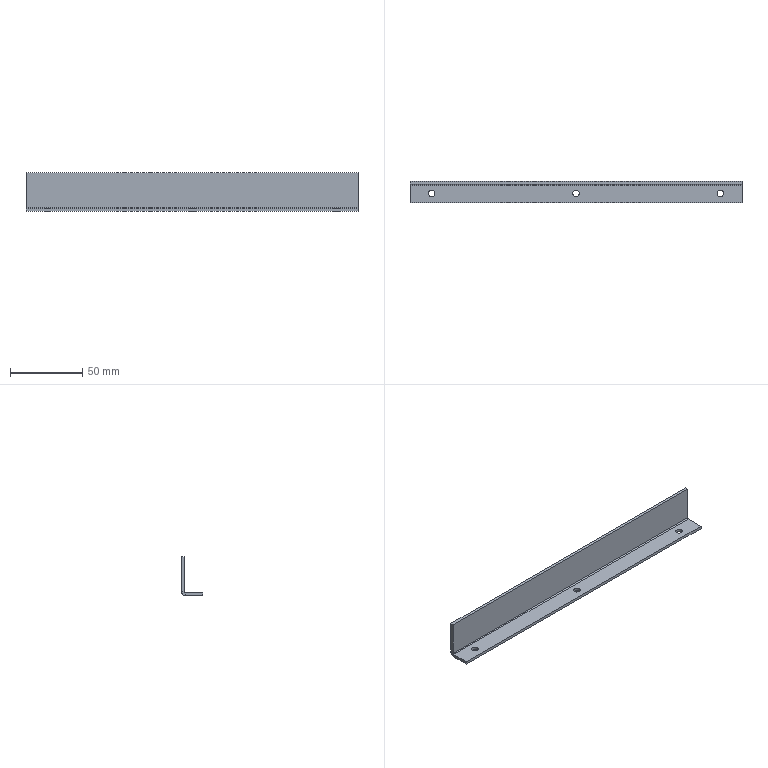Component | SolidWorks | P-SLJ-001-003-2 | 1 solid | 20 faces | box 230 x 15 x 27 mm | volume 17962 mm3 | plane 12 | cylinder 8 | commonest cylinder face diameters 4.5 x6 5.473 x1 1.473 x1 | material SUS 304
STEP:
#1=COLOUR_RGB('',0.7922,0.8196,0.9333);
#2=FILL_AREA_STYLE_COLOUR('',#1);
#3=FILL_AREA_STYLE('',(#2));
#4=SURFACE_STYLE_FILL_AREA(#3);
#5=SURFACE_SIDE_STYLE('',(#4));
#6=SURFACE_STYLE_USAGE(.BOTH.,#5);
#7=PRESENTATION_STYLE_ASSIGNMENT((#6));
#8=CARTESIAN_POINT('',(-1.801,-2.579,39.434));
#9=VERTEX_POINT('',#8);
#10=CARTESIAN_POINT('',(-1.624,-2.579,39.434));
#11=VERTEX_POINT('',#10);
#12=CARTESIAN_POINT('',(-1.713,-2.579,39.434));
#13=DIRECTION('',(0.,0.,1.));
#14=DIRECTION('',(1.,0.,0.));
#15=AXIS2_PLACEMENT_3D('',#12,#13,#14);
#16=CIRCLE('',#15,0.08858);
#17=EDGE_CURVE('',#9,#11,#16,.T.);
#18=ORIENTED_EDGE('',*,*,#17,.F.);
#19=CARTESIAN_POINT('',(-1.801,-2.579,39.513));
#20=VERTEX_POINT('',#19);
#21=CARTESIAN_POINT('',(-1.801,-2.579,39.513));
#22=DIRECTION('',(0.,0.,1.));
#23=VECTOR('',#22,39.37);
#24=LINE('',#21,#23);
#25=EDGE_CURVE('',#9,#20,#24,.T.);
#26=ORIENTED_EDGE('',*,*,#25,.T.);
#27=CARTESIAN_POINT('',(-1.624,-2.579,39.513));
#28=VERTEX_POINT('',#27);
#29=CARTESIAN_POINT('',(-1.713,-2.579,39.513));
#30=DIRECTION('',(0.,0.,1.));
#31=DIRECTION('',(1.,0.,0.));
#32=AXIS2_PLACEMENT_3D('',#29,#30,#31);
#33=CIRCLE('',#32,0.08858);
#34=EDGE_CURVE('',#20,#28,#33,.T.);
#35=ORIENTED_EDGE('',*,*,#34,.T.);
#36=CARTESIAN_POINT('',(-1.624,-2.579,39.513));
#37=DIRECTION('',(0.,0.,1.));
#38=VECTOR('',#37,39.37);
#39=LINE('',#36,#38);
#40=EDGE_CURVE('',#11,#28,#39,.T.);
#41=ORIENTED_EDGE('',*,*,#40,.F.);
#42=EDGE_LOOP('',(#18,#26,#35,#41));
#43=FACE_OUTER_BOUND('',#42,.T.);
#44=CARTESIAN_POINT('',(-1.713,-2.579,39.513));
#45=DIRECTION('',(0.,0.,1.));
#46=DIRECTION('',(1.,0.,0.));
#47=AXIS2_PLACEMENT_3D('',#44,#45,#46);
#48=CYLINDRICAL_SURFACE('',#47,0.08858);
#49=ADVANCED_FACE('',(#43),#48,.F.);
#50=CARTESIAN_POINT('',(2.136,-2.579,39.434));
#51=VERTEX_POINT('',#50);
#52=CARTESIAN_POINT('',(2.313,-2.579,39.434));
#53=VERTEX_POINT('',#52);
#54=CARTESIAN_POINT('',(2.224,-2.579,39.434));
#55=DIRECTION('',(0.,0.,1.));
#56=DIRECTION('',(1.,0.,0.));
#57=AXIS2_PLACEMENT_3D('',#54,#55,#56);
#58=CIRCLE('',#57,0.08858);
#59=EDGE_CURVE('',#51,#53,#58,.T.);
#60=ORIENTED_EDGE('',*,*,#59,.F.);
#61=CARTESIAN_POINT('',(2.136,-2.579,39.513));
#62=VERTEX_POINT('',#61);
#63=CARTESIAN_POINT('',(2.136,-2.579,39.513));
#64=DIRECTION('',(0.,0.,1.));
#65=VECTOR('',#64,39.37);
#66=LINE('',#63,#65);
#67=EDGE_CURVE('',#51,#62,#66,.T.);
#68=ORIENTED_EDGE('',*,*,#67,.T.);
#69=CARTESIAN_POINT('',(2.313,-2.579,39.513));
#70=VERTEX_POINT('',#69);
#71=CARTESIAN_POINT('',(2.224,-2.579,39.513));
#72=DIRECTION('',(0.,0.,1.));
#73=DIRECTION('',(1.,0.,0.));
#74=AXIS2_PLACEMENT_3D('',#71,#72,#73);
#75=CIRCLE('',#74,0.08858);
#76=EDGE_CURVE('',#62,#70,#75,.T.);
#77=ORIENTED_EDGE('',*,*,#76,.T.);
#78=CARTESIAN_POINT('',(2.313,-2.579,39.513));
#79=DIRECTION('',(0.,0.,1.));
#80=VECTOR('',#79,39.37);
#81=LINE('',#78,#80);
#82=EDGE_CURVE('',#53,#70,#81,.T.);
#83=ORIENTED_EDGE('',*,*,#82,.F.);
#84=EDGE_LOOP('',(#60,#68,#77,#83));
#85=FACE_OUTER_BOUND('',#84,.T.);
#86=CARTESIAN_POINT('',(2.224,-2.579,39.513));
#87=DIRECTION('',(0.,0.,1.));
#88=DIRECTION('',(1.,0.,0.));
#89=AXIS2_PLACEMENT_3D('',#86,#87,#88);
#90=CYLINDRICAL_SURFACE('',#89,0.08858);
#91=ADVANCED_FACE('',(#85),#90,.F.);
#92=CARTESIAN_POINT('',(6.073,-2.579,39.434));
#93=VERTEX_POINT('',#92);
#94=CARTESIAN_POINT('',(6.25,-2.579,39.434));
#95=VERTEX_POINT('',#94);
#96=CARTESIAN_POINT('',(6.161,-2.579,39.434));
#97=DIRECTION('',(0.,0.,1.));
#98=DIRECTION('',(1.,0.,0.));
#99=AXIS2_PLACEMENT_3D('',#96,#97,#98);
#100=CIRCLE('',#99,0.08858);
#101=EDGE_CURVE('',#93,#95,#100,.T.);
#102=ORIENTED_EDGE('',*,*,#101,.F.);
#103=CARTESIAN_POINT('',(6.073,-2.579,39.513));
#104=VERTEX_POINT('',#103);
#105=CARTESIAN_POINT('',(6.073,-2.579,39.513));
#106=DIRECTION('',(0.,0.,1.));
#107=VECTOR('',#106,39.37);
#108=LINE('',#105,#107);
#109=EDGE_CURVE('',#93,#104,#108,.T.);
#110=ORIENTED_EDGE('',*,*,#109,.T.);
#111=CARTESIAN_POINT('',(6.25,-2.579,39.513));
#112=VERTEX_POINT('',#111);
#113=CARTESIAN_POINT('',(6.161,-2.579,39.513));
#114=DIRECTION('',(0.,0.,1.));
#115=DIRECTION('',(1.,0.,0.));
#116=AXIS2_PLACEMENT_3D('',#113,#114,#115);
#117=CIRCLE('',#116,0.08858);
#118=EDGE_CURVE('',#104,#112,#117,.T.);
#119=ORIENTED_EDGE('',*,*,#118,.T.);
#120=CARTESIAN_POINT('',(6.25,-2.579,39.513));
#121=DIRECTION('',(0.,0.,1.));
#122=VECTOR('',#121,39.37);
#123=LINE('',#120,#122);
#124=EDGE_CURVE('',#95,#112,#123,.T.);
#125=ORIENTED_EDGE('',*,*,#124,.F.);
#126=EDGE_LOOP('',(#102,#110,#119,#125));
#127=FACE_OUTER_BOUND('',#126,.T.);
#128=CARTESIAN_POINT('',(6.161,-2.579,39.513));
#129=DIRECTION('',(0.,0.,1.));
#130=DIRECTION('',(1.,0.,0.));
#131=AXIS2_PLACEMENT_3D('',#128,#129,#130);
#132=CYLINDRICAL_SURFACE('',#131,0.08858);
#133=ADVANCED_FACE('',(#127),#132,.F.);
#134=CARTESIAN_POINT('',(-2.303,-2.352,39.513));
#135=VERTEX_POINT('',#134);
#136=CARTESIAN_POINT('',(-2.303,-2.835,39.513));
#137=VERTEX_POINT('',#136);
#138=CARTESIAN_POINT('',(-2.303,-2.835,39.513));
#139=DIRECTION('',(0.,-1.,0.));
#140=VECTOR('',#139,39.37);
#141=LINE('',#138,#140);
#142=EDGE_CURVE('',#135,#137,#141,.T.);
#143=ORIENTED_EDGE('',*,*,#142,.F.);
#144=CARTESIAN_POINT('',(-2.303,-2.352,39.434));
#145=VERTEX_POINT('',#144);
#146=CARTESIAN_POINT('',(-2.303,-2.352,39.513));
#147=DIRECTION('',(0.,0.,-1.));
#148=VECTOR('',#147,39.37);
#149=LINE('',#146,#148);
#150=EDGE_CURVE('',#135,#145,#149,.T.);
#151=ORIENTED_EDGE('',*,*,#150,.T.);
#152=CARTESIAN_POINT('',(-2.303,-2.835,39.434));
#153=VERTEX_POINT('',#152);
#154=CARTESIAN_POINT('',(-2.303,-2.835,39.434));
#155=DIRECTION('',(0.,-1.,0.));
#156=VECTOR('',#155,39.37);
#157=LINE('',#154,#156);
#158=EDGE_CURVE('',#145,#153,#157,.T.);
#159=ORIENTED_EDGE('',*,*,#158,.T.);
#160=CARTESIAN_POINT('',(-2.303,-2.835,39.434));
#161=DIRECTION('',(0.,0.,1.));
#162=VECTOR('',#161,39.37);
#163=LINE('',#160,#162);
#164=EDGE_CURVE('',#153,#137,#163,.T.);
#165=ORIENTED_EDGE('',*,*,#164,.T.);
#166=EDGE_LOOP('',(#143,#151,#159,#165));
#167=FACE_OUTER_BOUND('',#166,.T.);
#168=CARTESIAN_POINT('',(-2.303,-2.835,39.434));
#169=DIRECTION('',(-1.,0.,0.));
#170=DIRECTION('',(0.,0.,1.));
#171=AXIS2_PLACEMENT_3D('',#168,#169,#170);
#172=PLANE('',#171);
#173=ADVANCED_FACE('',(#167),#172,.T.);
#174=CARTESIAN_POINT('',(-1.713,-2.579,39.434));
#175=DIRECTION('',(0.,0.,1.));
#176=DIRECTION('',(1.,0.,0.));
#177=AXIS2_PLACEMENT_3D('',#174,#175,#176);
#178=CIRCLE('',#177,0.08858);
#179=EDGE_CURVE('',#11,#9,#178,.T.);
#180=ORIENTED_EDGE('',*,*,#179,.T.);
#181=ORIENTED_EDGE('',*,*,#17,.T.);
#182=EDGE_LOOP('',(#180,#181));
#183=FACE_BOUND('',#182,.T.);
#184=CARTESIAN_POINT('',(2.224,-2.579,39.434));
#185=DIRECTION('',(0.,0.,1.));
#186=DIRECTION('',(1.,0.,0.));
#187=AXIS2_PLACEMENT_3D('',#184,#185,#186);
#188=CIRCLE('',#187,0.08858);
#189=EDGE_CURVE('',#53,#51,#188,.T.);
#190=ORIENTED_EDGE('',*,*,#189,.T.);
#191=ORIENTED_EDGE('',*,*,#59,.T.);
#192=EDGE_LOOP('',(#190,#191));
#193=FACE_BOUND('',#192,.T.);
#194=CARTESIAN_POINT('',(6.161,-2.579,39.434));
#195=DIRECTION('',(0.,0.,1.));
#196=DIRECTION('',(1.,0.,0.));
#197=AXIS2_PLACEMENT_3D('',#194,#195,#196);
#198=CIRCLE('',#197,0.08858);
#199=EDGE_CURVE('',#95,#93,#198,.T.);
#200=ORIENTED_EDGE('',*,*,#199,.T.);
#201=ORIENTED_EDGE('',*,*,#101,.T.);
#202=EDGE_LOOP('',(#200,#201));
#203=FACE_BOUND('',#202,.T.);
#204=ORIENTED_EDGE('',*,*,#158,.F.);
#205=CARTESIAN_POINT('',(6.752,-2.352,39.434));
#206=VERTEX_POINT('',#205);
#207=CARTESIAN_POINT('',(-2.303,-2.352,39.434));
#208=DIRECTION('',(1.,0.,0.));
#209=VECTOR('',#208,39.37);
#210=LINE('',#207,#209);
#211=EDGE_CURVE('',#145,#206,#210,.T.);
#212=ORIENTED_EDGE('',*,*,#211,.T.);
#213=CARTESIAN_POINT('',(6.752,-2.835,39.434));
#214=VERTEX_POINT('',#213);
#215=CARTESIAN_POINT('',(6.752,-2.835,39.434));
#216=DIRECTION('',(-0.,1.,0.));
#217=VECTOR('',#216,39.37);
#218=LINE('',#215,#217);
#219=EDGE_CURVE('',#214,#206,#218,.T.);
#220=ORIENTED_EDGE('',*,*,#219,.F.);
#221=CARTESIAN_POINT('',(-2.303,-2.835,39.434));
#222=DIRECTION('',(1.,0.,0.));
#223=VECTOR('',#222,39.37);
#224=LINE('',#221,#223);
#225=EDGE_CURVE('',#153,#214,#224,.T.);
#226=ORIENTED_EDGE('',*,*,#225,.F.);
#227=EDGE_LOOP('',(#204,#212,#220,#226));
#228=FACE_OUTER_BOUND('',#227,.T.);
#229=CARTESIAN_POINT('',(2.224,-2.579,39.434));
#230=DIRECTION('',(0.,0.,-1.));
#231=DIRECTION('',(-1.,0.,0.));
#232=AXIS2_PLACEMENT_3D('',#229,#230,#231);
#233=PLANE('',#232);
#234=ADVANCED_FACE('',(#183,#193,#203,#228),#233,.T.);
#235=CARTESIAN_POINT('',(-1.713,-2.579,39.513));
#236=DIRECTION('',(0.,0.,1.));
#237=DIRECTION('',(1.,0.,0.));
#238=AXIS2_PLACEMENT_3D('',#235,#236,#237);
#239=CIRCLE('',#238,0.08858);
#240=EDGE_CURVE('',#28,#20,#239,.T.);
#241=ORIENTED_EDGE('',*,*,#240,.F.);
#242=ORIENTED_EDGE('',*,*,#34,.F.);
#243=EDGE_LOOP('',(#241,#242));
#244=FACE_BOUND('',#243,.T.);
#245=CARTESIAN_POINT('',(2.224,-2.579,39.513));
#246=DIRECTION('',(0.,0.,1.));
#247=DIRECTION('',(1.,0.,0.));
#248=AXIS2_PLACEMENT_3D('',#245,#246,#247);
#249=CIRCLE('',#248,0.08858);
#250=EDGE_CURVE('',#70,#62,#249,.T.);
#251=ORIENTED_EDGE('',*,*,#250,.F.);
#252=ORIENTED_EDGE('',*,*,#76,.F.);
#253=EDGE_LOOP('',(#251,#252));
#254=FACE_BOUND('',#253,.T.);
#255=CARTESIAN_POINT('',(6.161,-2.579,39.513));
#256=DIRECTION('',(0.,0.,1.));
#257=DIRECTION('',(1.,0.,0.));
#258=AXIS2_PLACEMENT_3D('',#255,#256,#257);
#259=CIRCLE('',#258,0.08858);
#260=EDGE_CURVE('',#112,#104,#259,.T.);
#261=ORIENTED_EDGE('',*,*,#260,.F.);
#262=ORIENTED_EDGE('',*,*,#118,.F.);
#263=EDGE_LOOP('',(#261,#262));
#264=FACE_BOUND('',#263,.T.);
#265=CARTESIAN_POINT('',(6.752,-2.352,39.513));
#266=VERTEX_POINT('',#265);
#267=CARTESIAN_POINT('',(-2.303,-2.352,39.513));
#268=DIRECTION('',(1.,0.,0.));
#269=VECTOR('',#268,39.37);
#270=LINE('',#267,#269);
#271=EDGE_CURVE('',#135,#266,#270,.T.);
#272=ORIENTED_EDGE('',*,*,#271,.F.);
#273=ORIENTED_EDGE('',*,*,#142,.T.);
#274=CARTESIAN_POINT('',(6.752,-2.835,39.513));
#275=VERTEX_POINT('',#274);
#276=CARTESIAN_POINT('',(-2.303,-2.835,39.513));
#277=DIRECTION('',(1.,0.,0.));
#278=VECTOR('',#277,39.37);
#279=LINE('',#276,#278);
#280=EDGE_CURVE('',#137,#275,#279,.T.);
#281=ORIENTED_EDGE('',*,*,#280,.T.);
#282=CARTESIAN_POINT('',(6.752,-2.835,39.513));
#283=DIRECTION('',(-0.,1.,0.));
#284=VECTOR('',#283,39.37);
#285=LINE('',#282,#284);
#286=EDGE_CURVE('',#275,#266,#285,.T.);
#287=ORIENTED_EDGE('',*,*,#286,.T.);
#288=EDGE_LOOP('',(#272,#273,#281,#287));
#289=FACE_OUTER_BOUND('',#288,.T.);
#290=CARTESIAN_POINT('',(2.224,-2.579,39.513));
#291=DIRECTION('',(0.,0.,-1.));
#292=DIRECTION('',(-1.,0.,0.));
#293=AXIS2_PLACEMENT_3D('',#290,#291,#292);
#294=PLANE('',#293);
#295=ADVANCED_FACE('',(#244,#254,#264,#289),#294,.F.);
#296=CARTESIAN_POINT('',(6.752,-2.352,39.513));
#297=DIRECTION('',(0.,0.,-1.));
#298=VECTOR('',#297,39.37);
#299=LINE('',#296,#298);
#300=EDGE_CURVE('',#266,#206,#299,.T.);
#301=ORIENTED_EDGE('',*,*,#300,.F.);
#302=ORIENTED_EDGE('',*,*,#286,.F.);
#303=CARTESIAN_POINT('',(6.752,-2.835,39.434));
#304=DIRECTION('',(0.,0.,1.));
#305=VECTOR('',#304,39.37);
#306=LINE('',#303,#305);
#307=EDGE_CURVE('',#214,#275,#306,.T.);
#308=ORIENTED_EDGE('',*,*,#307,.F.);
#309=ORIENTED_EDGE('',*,*,#219,.T.);
#310=EDGE_LOOP('',(#301,#302,#308,#309));
#311=FACE_OUTER_BOUND('',#310,.T.);
#312=CARTESIAN_POINT('',(6.752,-2.835,39.434));
#313=DIRECTION('',(1.,0.,0.));
#314=DIRECTION('',(0.,0.,-1.));
#315=AXIS2_PLACEMENT_3D('',#312,#313,#314);
#316=PLANE('',#315);
#317=ADVANCED_FACE('',(#311),#316,.T.);
#318=ORIENTED_EDGE('',*,*,#280,.F.);
#319=ORIENTED_EDGE('',*,*,#164,.F.);
#320=ORIENTED_EDGE('',*,*,#225,.T.);
#321=ORIENTED_EDGE('',*,*,#307,.T.);
#322=EDGE_LOOP('',(#318,#319,#320,#321));
#323=FACE_OUTER_BOUND('',#322,.T.);
#324=CARTESIAN_POINT('',(-2.303,-2.835,39.434));
#325=DIRECTION('',(0.,-1.,0.));
#326=DIRECTION('',(1.,0.,0.));
#327=AXIS2_PLACEMENT_3D('',#324,#325,#326);
#328=PLANE('',#327);
#329=ADVANCED_FACE('',(#323),#328,.T.);
#330=CARTESIAN_POINT('',(6.752,-2.323,39.542));
#331=VERTEX_POINT('',#330);
#332=CARTESIAN_POINT('',(6.752,-2.244,39.542));
#333=VERTEX_POINT('',#332);
#334=CARTESIAN_POINT('',(6.752,-2.323,39.542));
#335=DIRECTION('',(-0.,1.,-0.));
#336=VECTOR('',#335,39.37);
#337=LINE('',#334,#336);
#338=EDGE_CURVE('',#331,#333,#337,.T.);
#339=ORIENTED_EDGE('',*,*,#338,.F.);
#340=CARTESIAN_POINT('',(6.752,-2.352,39.542));
#341=DIRECTION('',(1.,0.,0.));
#342=DIRECTION('',(0.,0.,1.));
#343=AXIS2_PLACEMENT_3D('',#340,#341,#342);
#344=CIRCLE('',#343,0.029);
#345=EDGE_CURVE('',#266,#331,#344,.T.);
#346=ORIENTED_EDGE('',*,*,#345,.F.);
#347=ORIENTED_EDGE('',*,*,#300,.T.);
#348=CARTESIAN_POINT('',(6.752,-2.352,39.542));
#349=DIRECTION('',(1.,0.,0.));
#350=DIRECTION('',(0.,0.,1.));
#351=AXIS2_PLACEMENT_3D('',#348,#349,#350);
#352=CIRCLE('',#351,0.1077);
#353=EDGE_CURVE('',#206,#333,#352,.T.);
#354=ORIENTED_EDGE('',*,*,#353,.T.);
#355=EDGE_LOOP('',(#339,#346,#347,#354));
#356=FACE_OUTER_BOUND('',#355,.T.);
#357=CARTESIAN_POINT('',(6.752,-2.352,39.542));
#358=DIRECTION('',(1.,0.,0.));
#359=DIRECTION('',(0.,0.,-1.));
#360=AXIS2_PLACEMENT_3D('',#357,#358,#359);
#361=PLANE('',#360);
#362=ADVANCED_FACE('',(#356),#361,.T.);
#363=CARTESIAN_POINT('',(-2.303,-2.323,39.542));
#364=VERTEX_POINT('',#363);
#365=CARTESIAN_POINT('',(-2.303,-2.352,39.542));
#366=DIRECTION('',(-1.,0.,0.));
#367=DIRECTION('',(0.,0.,1.));
#368=AXIS2_PLACEMENT_3D('',#365,#366,#367);
#369=CIRCLE('',#368,0.029);
#370=EDGE_CURVE('',#364,#135,#369,.T.);
#371=ORIENTED_EDGE('',*,*,#370,.F.);
#372=CARTESIAN_POINT('',(-2.303,-2.244,39.542));
#373=VERTEX_POINT('',#372);
#374=CARTESIAN_POINT('',(-2.303,-2.323,39.542));
#375=DIRECTION('',(-0.,1.,-0.));
#376=VECTOR('',#375,39.37);
#377=LINE('',#374,#376);
#378=EDGE_CURVE('',#364,#373,#377,.T.);
#379=ORIENTED_EDGE('',*,*,#378,.T.);
#380=CARTESIAN_POINT('',(-2.303,-2.352,39.542));
#381=DIRECTION('',(-1.,0.,0.));
#382=DIRECTION('',(0.,0.,1.));
#383=AXIS2_PLACEMENT_3D('',#380,#381,#382);
#384=CIRCLE('',#383,0.1077);
#385=EDGE_CURVE('',#373,#145,#384,.T.);
#386=ORIENTED_EDGE('',*,*,#385,.T.);
#387=ORIENTED_EDGE('',*,*,#150,.F.);
#388=EDGE_LOOP('',(#371,#379,#386,#387));
#389=FACE_OUTER_BOUND('',#388,.T.);
#390=CARTESIAN_POINT('',(-2.303,-2.352,39.542));
#391=DIRECTION('',(1.,0.,0.));
#392=DIRECTION('',(0.,0.,-1.));
#393=AXIS2_PLACEMENT_3D('',#390,#391,#392);
#394=PLANE('',#393);
#395=ADVANCED_FACE('',(#389),#394,.F.);
#396=ORIENTED_EDGE('',*,*,#211,.F.);
#397=ORIENTED_EDGE('',*,*,#385,.F.);
#398=CARTESIAN_POINT('',(2.224,-2.244,39.542));
#399=DIRECTION('',(1.,-0.,-0.));
#400=VECTOR('',#399,39.37);
#401=LINE('',#398,#400);
#402=EDGE_CURVE('',#373,#333,#401,.T.);
#403=ORIENTED_EDGE('',*,*,#402,.T.);
#404=ORIENTED_EDGE('',*,*,#353,.F.);
#405=EDGE_LOOP('',(#396,#397,#403,#404));
#406=FACE_OUTER_BOUND('',#405,.T.);
#407=CARTESIAN_POINT('',(-2.303,-2.352,39.542));
#408=DIRECTION('',(-1.,0.,0.));
#409=DIRECTION('',(0.,1.,0.));
#410=AXIS2_PLACEMENT_3D('',#407,#408,#409);
#411=CYLINDRICAL_SURFACE('',#410,0.1077);
#412=ADVANCED_FACE('',(#406),#411,.T.);
#413=ORIENTED_EDGE('',*,*,#271,.T.);
#414=ORIENTED_EDGE('',*,*,#345,.T.);
#415=CARTESIAN_POINT('',(6.752,-2.323,39.542));
#416=DIRECTION('',(-1.,0.,0.));
#417=VECTOR('',#416,39.37);
#418=LINE('',#415,#417);
#419=EDGE_CURVE('',#331,#364,#418,.T.);
#420=ORIENTED_EDGE('',*,*,#419,.T.);
#421=ORIENTED_EDGE('',*,*,#370,.T.);
#422=EDGE_LOOP('',(#413,#414,#420,#421));
#423=FACE_OUTER_BOUND('',#422,.T.);
#424=CARTESIAN_POINT('',(-2.303,-2.352,39.542));
#425=DIRECTION('',(-1.,0.,0.));
#426=DIRECTION('',(0.,1.,0.));
#427=AXIS2_PLACEMENT_3D('',#424,#425,#426);
#428=CYLINDRICAL_SURFACE('',#427,0.029);
#429=ADVANCED_FACE('',(#423),#428,.F.);
#430=ORIENTED_EDGE('',*,*,#378,.F.);
#431=CARTESIAN_POINT('',(-2.303,-2.323,40.497));
#432=VERTEX_POINT('',#431);
#433=CARTESIAN_POINT('',(-2.303,-2.323,40.497));
#434=DIRECTION('',(-0.,0.,1.));
#435=VECTOR('',#434,39.37);
#436=LINE('',#433,#435);
#437=EDGE_CURVE('',#364,#432,#436,.T.);
#438=ORIENTED_EDGE('',*,*,#437,.T.);
#439=CARTESIAN_POINT('',(-2.303,-2.244,40.497));
#440=VERTEX_POINT('',#439);
#441=CARTESIAN_POINT('',(-2.303,-2.244,40.497));
#442=DIRECTION('',(0.,-1.,0.));
#443=VECTOR('',#442,39.37);
#444=LINE('',#441,#443);
#445=EDGE_CURVE('',#440,#432,#444,.T.);
#446=ORIENTED_EDGE('',*,*,#445,.F.);
#447=CARTESIAN_POINT('',(-2.303,-2.244,40.497));
#448=DIRECTION('',(-0.,0.,1.));
#449=VECTOR('',#448,39.37);
#450=LINE('',#447,#449);
#451=EDGE_CURVE('',#373,#440,#450,.T.);
#452=ORIENTED_EDGE('',*,*,#451,.F.);
#453=EDGE_LOOP('',(#430,#438,#446,#452));
#454=FACE_OUTER_BOUND('',#453,.T.);
#455=CARTESIAN_POINT('',(-2.303,-2.244,40.497));
#456=DIRECTION('',(1.,0.,0.));
#457=DIRECTION('',(0.,0.,-1.));
#458=AXIS2_PLACEMENT_3D('',#455,#456,#457);
#459=PLANE('',#458);
#460=ADVANCED_FACE('',(#454),#459,.F.);
#461=ORIENTED_EDGE('',*,*,#338,.T.);
#462=CARTESIAN_POINT('',(6.752,-2.244,40.497));
#463=VERTEX_POINT('',#462);
#464=CARTESIAN_POINT('',(6.752,-2.244,39.513));
#465=DIRECTION('',(0.,-0.,-1.));
#466=VECTOR('',#465,39.37);
#467=LINE('',#464,#466);
#468=EDGE_CURVE('',#463,#333,#467,.T.);
#469=ORIENTED_EDGE('',*,*,#468,.F.);
#470=CARTESIAN_POINT('',(6.752,-2.323,40.497));
#471=VERTEX_POINT('',#470);
#472=CARTESIAN_POINT('',(6.752,-2.244,40.497));
#473=DIRECTION('',(0.,-1.,0.));
#474=VECTOR('',#473,39.37);
#475=LINE('',#472,#474);
#476=EDGE_CURVE('',#463,#471,#475,.T.);
#477=ORIENTED_EDGE('',*,*,#476,.T.);
#478=CARTESIAN_POINT('',(6.752,-2.323,39.513));
#479=DIRECTION('',(0.,-0.,-1.));
#480=VECTOR('',#479,39.37);
#481=LINE('',#478,#480);
#482=EDGE_CURVE('',#471,#331,#481,.T.);
#483=ORIENTED_EDGE('',*,*,#482,.T.);
#484=EDGE_LOOP('',(#461,#469,#477,#483));
#485=FACE_OUTER_BOUND('',#484,.T.);
#486=CARTESIAN_POINT('',(6.752,-2.244,39.513));
#487=DIRECTION('',(-1.,0.,0.));
#488=DIRECTION('',(0.,0.,1.));
#489=AXIS2_PLACEMENT_3D('',#486,#487,#488);
#490=PLANE('',#489);
#491=ADVANCED_FACE('',(#485),#490,.F.);
#492=ORIENTED_EDGE('',*,*,#402,.F.);
#493=ORIENTED_EDGE('',*,*,#451,.T.);
#494=CARTESIAN_POINT('',(6.752,-2.244,40.497));
#495=DIRECTION('',(1.,0.,0.));
#496=VECTOR('',#495,39.37);
#497=LINE('',#494,#496);
#498=EDGE_CURVE('',#440,#463,#497,.T.);
#499=ORIENTED_EDGE('',*,*,#498,.T.);
#500=ORIENTED_EDGE('',*,*,#468,.T.);
#501=EDGE_LOOP('',(#492,#493,#499,#500));
#502=FACE_OUTER_BOUND('',#501,.T.);
#503=CARTESIAN_POINT('',(2.224,-2.244,39.513));
#504=DIRECTION('',(0.,-1.,0.));
#505=DIRECTION('',(-0.,0.,1.));
#506=AXIS2_PLACEMENT_3D('',#503,#504,#505);
#507=PLANE('',#506);
#508=ADVANCED_FACE('',(#502),#507,.F.);
#509=ORIENTED_EDGE('',*,*,#437,.F.);
#510=ORIENTED_EDGE('',*,*,#419,.F.);
#511=ORIENTED_EDGE('',*,*,#482,.F.);
#512=CARTESIAN_POINT('',(6.752,-2.323,40.497));
#513=DIRECTION('',(1.,0.,0.));
#514=VECTOR('',#513,39.37);
#515=LINE('',#512,#514);
#516=EDGE_CURVE('',#432,#471,#515,.T.);
#517=ORIENTED_EDGE('',*,*,#516,.F.);
#518=EDGE_LOOP('',(#509,#510,#511,#517));
#519=FACE_OUTER_BOUND('',#518,.T.);
#520=CARTESIAN_POINT('',(2.224,-2.323,39.513));
#521=DIRECTION('',(0.,-1.,0.));
#522=DIRECTION('',(-0.,0.,1.));
#523=AXIS2_PLACEMENT_3D('',#520,#521,#522);
#524=PLANE('',#523);
#525=ADVANCED_FACE('',(#519),#524,.T.);
#526=ORIENTED_EDGE('',*,*,#516,.T.);
#527=ORIENTED_EDGE('',*,*,#476,.F.);
#528=ORIENTED_EDGE('',*,*,#498,.F.);
#529=ORIENTED_EDGE('',*,*,#445,.T.);
#530=EDGE_LOOP('',(#526,#527,#528,#529));
#531=FACE_OUTER_BOUND('',#530,.T.);
#532=CARTESIAN_POINT('',(6.752,-2.244,40.497));
#533=DIRECTION('',(0.,-0.,-1.));
#534=DIRECTION('',(0.,-1.,0.));
#535=AXIS2_PLACEMENT_3D('',#532,#533,#534);
#536=PLANE('',#535);
#537=ADVANCED_FACE('',(#531),#536,.F.);
#538=ORIENTED_EDGE('',*,*,#109,.F.);
#539=ORIENTED_EDGE('',*,*,#199,.F.);
#540=ORIENTED_EDGE('',*,*,#124,.T.);
#541=ORIENTED_EDGE('',*,*,#260,.T.);
#542=EDGE_LOOP('',(#538,#539,#540,#541));
#543=FACE_OUTER_BOUND('',#542,.T.);
#544=CARTESIAN_POINT('',(6.161,-2.579,39.513));
#545=DIRECTION('',(0.,0.,1.));
#546=DIRECTION('',(1.,0.,0.));
#547=AXIS2_PLACEMENT_3D('',#544,#545,#546);
#548=CYLINDRICAL_SURFACE('',#547,0.08858);
#549=ADVANCED_FACE('',(#543),#548,.F.);
#550=ORIENTED_EDGE('',*,*,#67,.F.);
#551=ORIENTED_EDGE('',*,*,#189,.F.);
#552=ORIENTED_EDGE('',*,*,#82,.T.);
#553=ORIENTED_EDGE('',*,*,#250,.T.);
#554=EDGE_LOOP('',(#550,#551,#552,#553));
#555=FACE_OUTER_BOUND('',#554,.T.);
#556=CARTESIAN_POINT('',(2.224,-2.579,39.513));
#557=DIRECTION('',(0.,0.,1.));
#558=DIRECTION('',(1.,0.,0.));
#559=AXIS2_PLACEMENT_3D('',#556,#557,#558);
#560=CYLINDRICAL_SURFACE('',#559,0.08858);
#561=ADVANCED_FACE('',(#555),#560,.F.);
#562=ORIENTED_EDGE('',*,*,#25,.F.);
#563=ORIENTED_EDGE('',*,*,#179,.F.);
#564=ORIENTED_EDGE('',*,*,#40,.T.);
#565=ORIENTED_EDGE('',*,*,#240,.T.);
#566=EDGE_LOOP('',(#562,#563,#564,#565));
#567=FACE_OUTER_BOUND('',#566,.T.);
#568=CARTESIAN_POINT('',(-1.713,-2.579,39.513));
#569=DIRECTION('',(0.,0.,1.));
#570=DIRECTION('',(1.,0.,0.));
#571=AXIS2_PLACEMENT_3D('',#568,#569,#570);
#572=CYLINDRICAL_SURFACE('',#571,0.08858);
#573=ADVANCED_FACE('',(#567),#572,.F.);
#574=CLOSED_SHELL('',(#49,#91,#133,#173,#234,#295,#317,#329,#362,#395,#412,#429,#460,#491,#508,#525,#537,#549,#561,#573));
#575=MANIFOLD_SOLID_BREP('',#574);
#576=STYLED_ITEM('',(#7),#575);
#577=(LENGTH_UNIT()NAMED_UNIT(*)SI_UNIT($,.METRE.));
#578=LENGTH_MEASURE_WITH_UNIT(LENGTH_MEASURE(0.0254),#577);
#579=DIMENSIONAL_EXPONENTS(1.,0.,0.,0.,0.,0.,0.);
#580=(CONVERSION_BASED_UNIT('',#578)LENGTH_UNIT()NAMED_UNIT(#579));
#581=UNCERTAINTY_MEASURE_WITH_UNIT(LENGTH_MEASURE(0.00001),#580,'','');
#582=(NAMED_UNIT(*)PLANE_ANGLE_UNIT()SI_UNIT($,.RADIAN.));
#583=(NAMED_UNIT(*)SI_UNIT($,.STERADIAN.)SOLID_ANGLE_UNIT());
#584=(GEOMETRIC_REPRESENTATION_CONTEXT(3)GLOBAL_UNCERTAINTY_ASSIGNED_CONTEXT((#581))GLOBAL_UNIT_ASSIGNED_CONTEXT((#580,#582,#583))REPRESENTATION_CONTEXT('',''));
#585=MECHANICAL_DESIGN_GEOMETRIC_PRESENTATION_REPRESENTATION('',(#576),#584);
#586=CARTESIAN_POINT('',(0.,0.,0.));
#587=DIRECTION('',(0.,0.,1.));
#588=DIRECTION('',(1.,0.,0.));
#589=AXIS2_PLACEMENT_3D('',#586,#587,#588);
#590=(LENGTH_UNIT()NAMED_UNIT(*)SI_UNIT($,.METRE.));
#591=LENGTH_MEASURE_WITH_UNIT(LENGTH_MEASURE(0.0254),#590);
#592=DIMENSIONAL_EXPONENTS(1.,0.,0.,0.,0.,0.,0.);
#593=(CONVERSION_BASED_UNIT('',#591)LENGTH_UNIT()NAMED_UNIT(#592));
#594=UNCERTAINTY_MEASURE_WITH_UNIT(LENGTH_MEASURE(0.00001),#593,'','');
#595=(NAMED_UNIT(*)PLANE_ANGLE_UNIT()SI_UNIT($,.RADIAN.));
#596=(NAMED_UNIT(*)SI_UNIT($,.STERADIAN.)SOLID_ANGLE_UNIT());
#597=(GEOMETRIC_REPRESENTATION_CONTEXT(3)GLOBAL_UNCERTAINTY_ASSIGNED_CONTEXT((#594))GLOBAL_UNIT_ASSIGNED_CONTEXT((#593,#595,#596))REPRESENTATION_CONTEXT('',''));
#598=ADVANCED_BREP_SHAPE_REPRESENTATION('',(#575,#589),#597);
#599=PRESENTATION_LAYER_ASSIGNMENT('','',(#576));